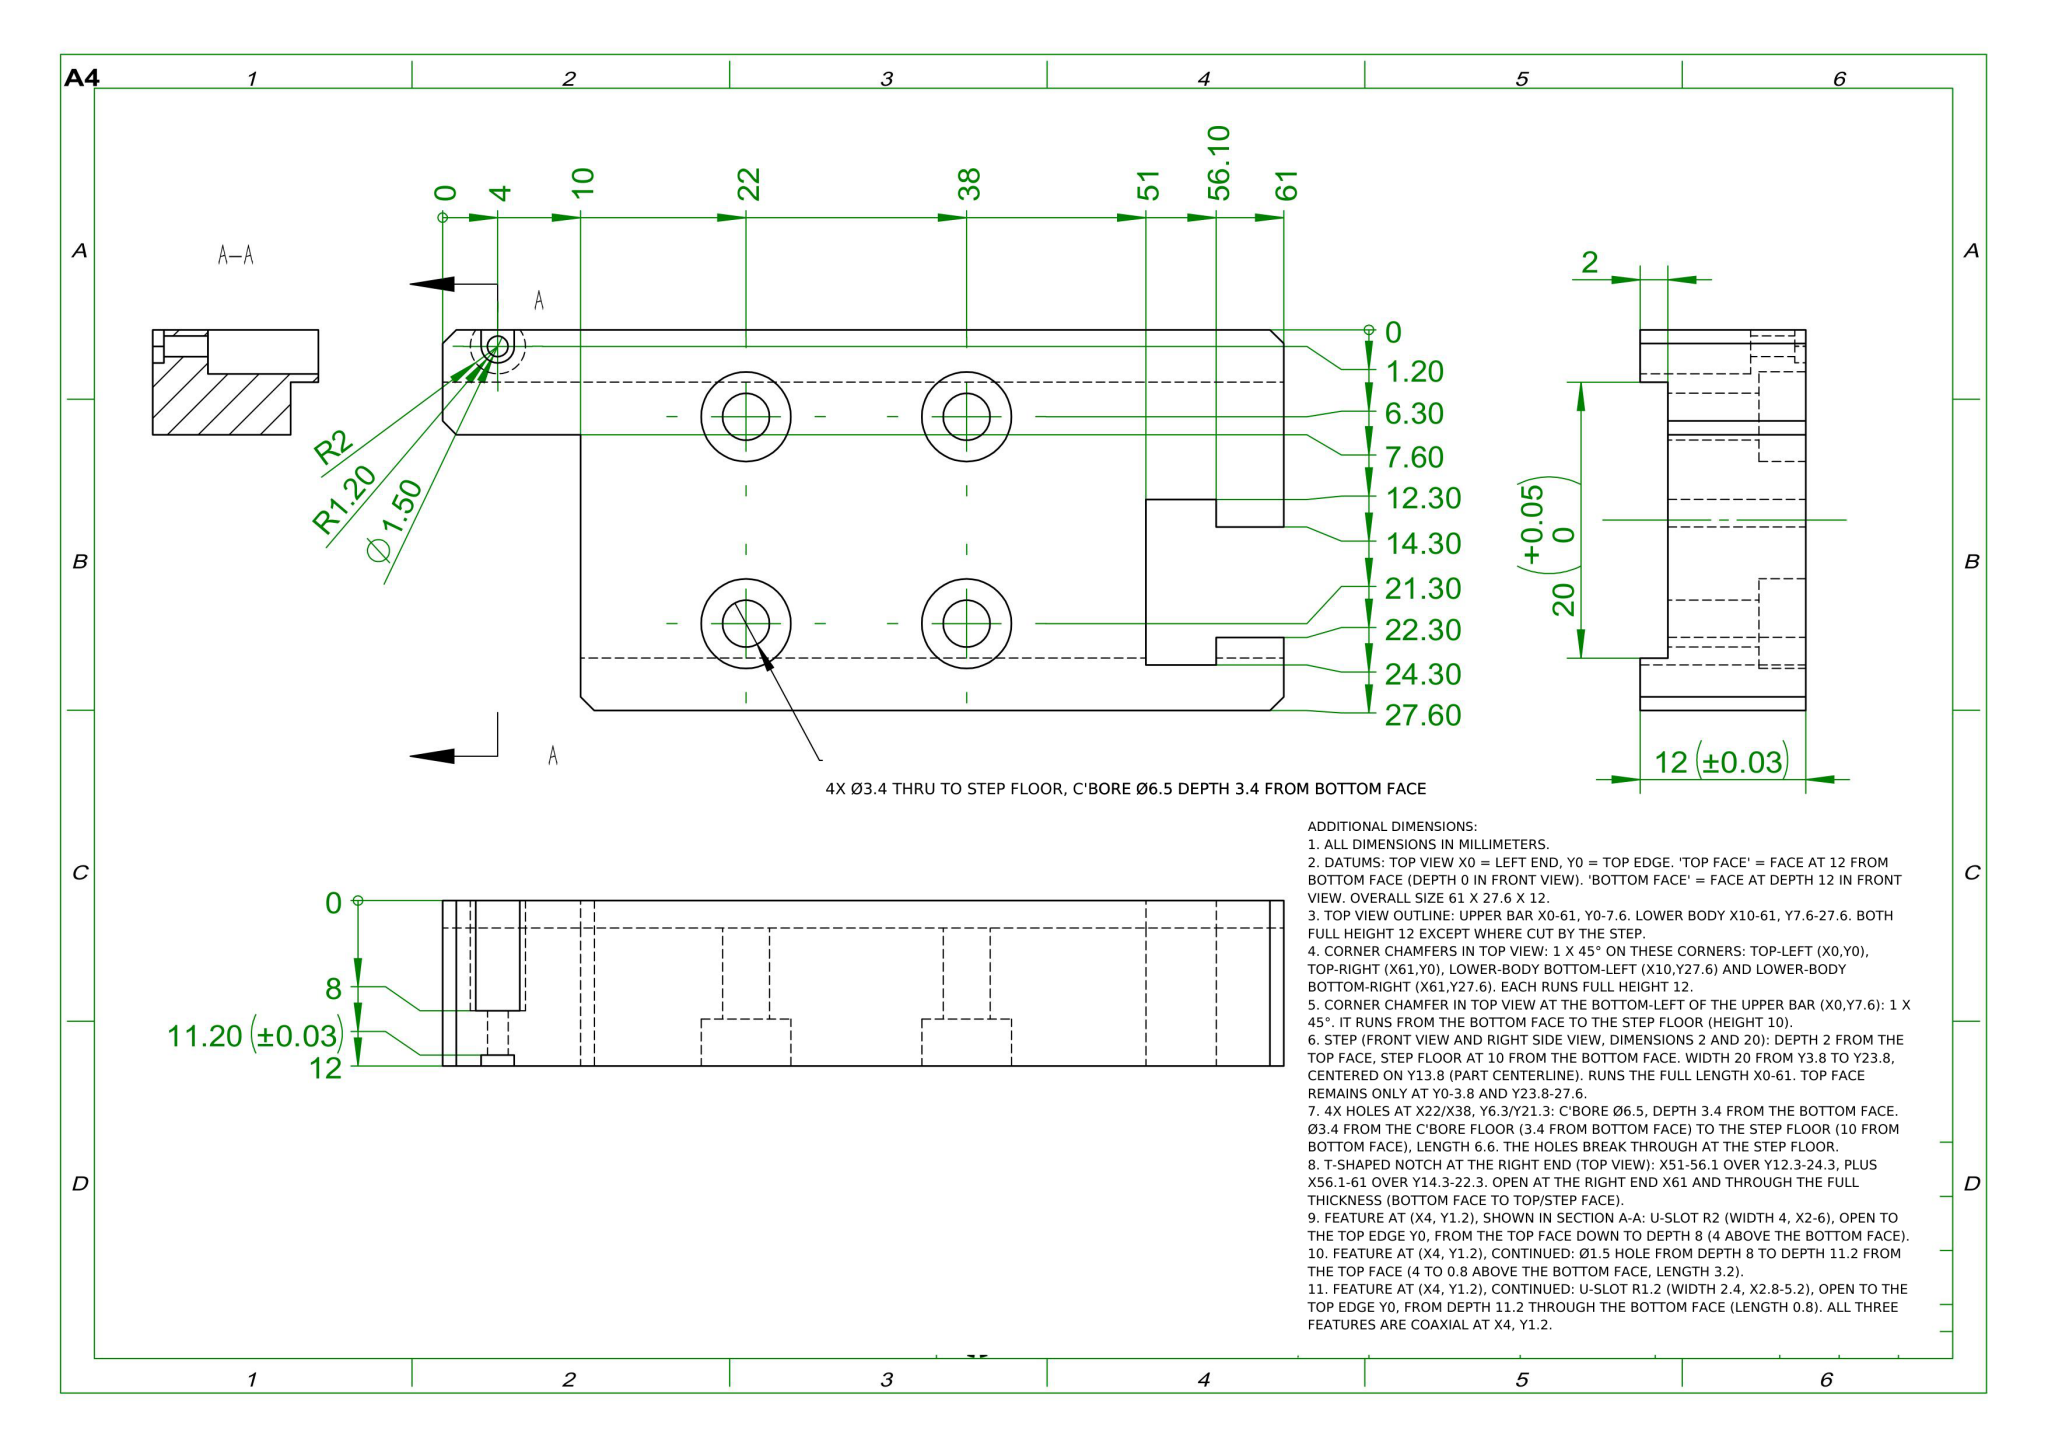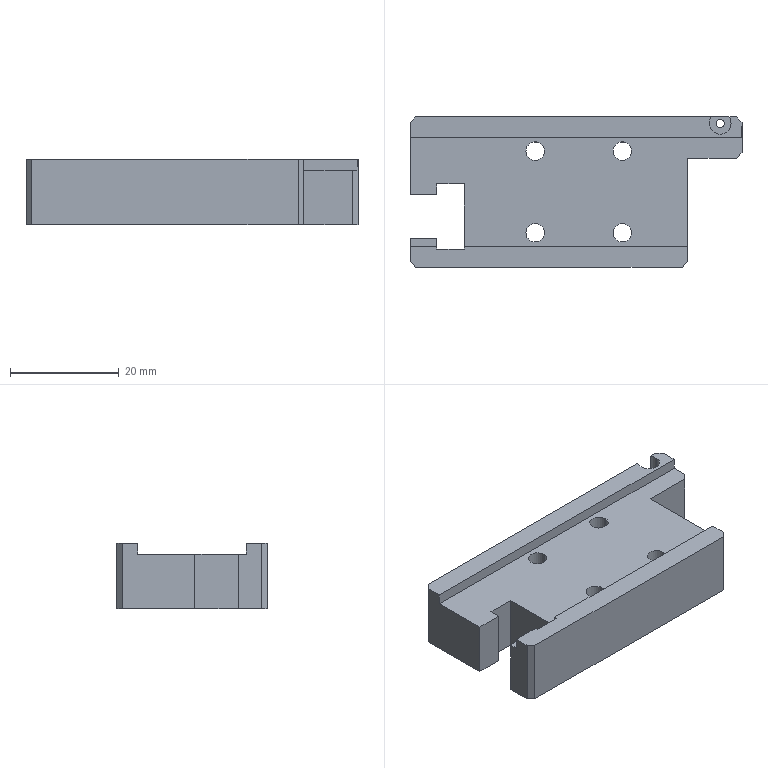Part | NX | mm | 1 solid | 57 faces | box 61 x 27.6 x 12 mm | volume 13862 mm3 | plane 35 | cylinder 22 | commonest cylinder face diameters 6.5 x8 3.4 x8 4 x3 1.5 x2 2.4 x1